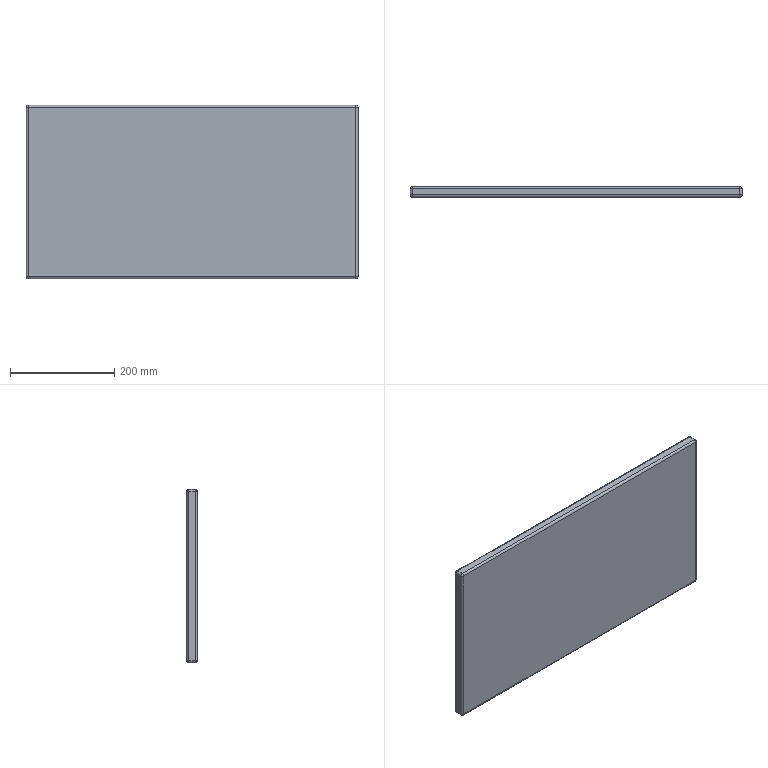Component | SolidWorks | AX00-100.1.1-1_23.1.1-1 | 1 solid | 26 faces | box 638 x 20 x 333 mm | volume 4235555 mm3 | cylinder 12 | sphere 8 | plane 6 | commonest cylinder face diameters 8 x12
build123d program:
from build123d import *

# Parameters (mm, degrees)
SKETCH1_W           = 638
SKETCH1_H           = 333
BOSS_EXTRUDE1_DEPTH = 10
FILLET1_R           = 4
FILLET2_R           = 4


with BuildPart() as part:
    # Sketch1 → Boss-Extrude1 (new, symmetric)
    with BuildSketch(Plane.XY):
        Rectangle(SKETCH1_W, SKETCH1_H)
    extrude(amount=BOSS_EXTRUDE1_DEPTH, both=True)

    # Fillet1
    fillet1_edges = [part.edges().sort_by_distance(p)[0] for p in [
        (319, -166.5, 0),
        (-319, -166.5, 0),
        (-319, 166.5, 0),
        (319, 166.5, 0),
    ]]
    fillet(fillet1_edges, radius=FILLET1_R)

    # Fillet2
    fillet2_edges = [part.edges().sort_by_distance(p)[0] for p in [
        (0, -166.5, -10),
        (0, -166.5, 10),
        (319, 0, -10),
        (-319, 0, -10),
        (0, 166.5, -10),
        (317.828, 165.328, -10),
        (317.828, -165.328, -10),
        (-317.828, 165.328, -10),
        (-317.828, -165.328, -10),
        (-319, 0, 10),
        (319, 0, 10),
        (0, 166.5, 10),
        (317.828, 165.328, 10),
        (317.828, -165.328, 10),
        (-317.828, 165.328, 10),
        (-317.828, -165.328, 10),
    ]]
    fillet(fillet2_edges, radius=FILLET2_R)


solid = part.part

# Placed as in the assembly
solid = solid.moved(Location((228.631, 1138.364, -4), (90, 0, 0)))